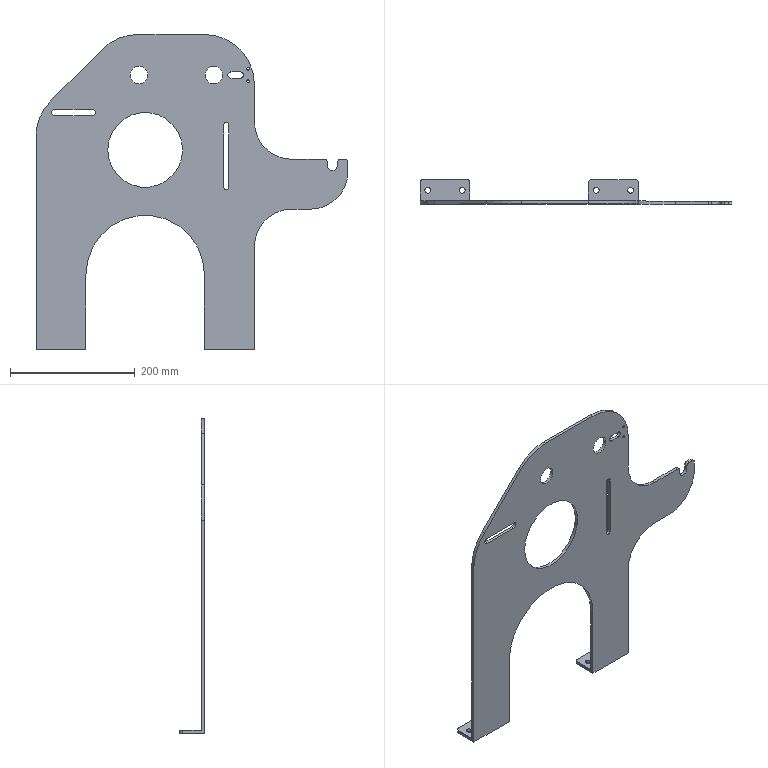Component | SolidWorks | VerticalPlate_Default_ByProcessing-3 | 1 solid | 72 faces | box 500 x 40 x 505 mm | volume 665775 mm3 | cylinder 41 | plane 27 | cone 4 | commonest cylinder face diameters 10 x13 9.225 x8 120 x5 4.2 x4 28 x4 160 x3 8 x2 16 x1
build123d program:
from build123d import *

# Parameters (mm, degrees)
SKETCH1_W                   = 350
SKETCH1_H                   = 500
BOSS_EXTRUDE1_DEPTH         = 2.5
SKETCH2_W                   = 150
SKETCH2_H                   = 80
BOSS_EXTRUDE2_DEPTH         = 5
SKETCH3_W                   = 350
SKETCH3_H                   = 40
BOSS_EXTRUDE3_DEPTH         = 5
CUT_EXTRUDE1_DEPTH          = 415.578
SKETCH6_R                   = 4.09
CUT_EXTRUDE3_DEPTH          = 598.521
SKETCH7_R                   = 60
CUT_EXTRUDE4_DEPTH          = 416.03
CHAMFER1_SIZE               = 130
FILLET2_R                   = 60
FILLET3_R                   = 80
SKETCH8_R                   = 14
CUT_EXTRUDE5_DEPTH          = 415.578
M5_TAPPED_HOLE1_D           = 4.2
M5_TAPPED_HOLE1_CSINK_D     = 5.05
M5_TAPPED_HOLE1_CSINK_ANGLE = 90
FILLET1_R                   = 5
SKETCH11_R                  = 4.613
CUT_EXTRUDE6_DEPTH          = 598.521
FILLET4_R                   = 60


with BuildPart() as part:
    # Sketch1 → Boss-Extrude1 (new, symmetric)
    with BuildSketch(Plane.XY):
        Rectangle(SKETCH1_W, SKETCH1_H)
    extrude(amount=BOSS_EXTRUDE1_DEPTH, both=True)

    # Sketch2 → Boss-Extrude2 (add)
    with BuildSketch(Plane.XY.offset(2.5)):
        with Locations((-250, 10)):
            Rectangle(SKETCH2_W, SKETCH2_H)
    extrude(amount=-BOSS_EXTRUDE2_DEPTH)

    # Sketch3 → Boss-Extrude3 (add)
    with BuildSketch(Plane.XZ.offset(250)):
        with Locations((0, 17.5)):
            Rectangle(SKETCH3_W, SKETCH3_H)
    extrude(amount=BOSS_EXTRUDE3_DEPTH)

    # Sketch4 → Cut-Extrude1 (cut, through all)
    with BuildSketch(Plane.XY.offset(2.5)):
        with BuildLine():
            Line((-292, 60), (-292, 40))
            ThreePointArc((-292, 40), (-300, 32), (-308, 40))
            Line((-308, 40), (-308, 60))
            ThreePointArc((-308, 60), (-300, 68), (-292, 60))
        make_face()
    extrude(amount=-CUT_EXTRUDE1_DEPTH, mode=Mode.SUBTRACT)

    # Sketch6 → Cut-Extrude3 (cut, through all)
    with BuildSketch(Plane(origin=(0, -250, 0), x_dir=(1, 0, 0), z_dir=(0, 1, 0))):
        with Locations(Location((-11.628, -27.97, 0), (0, 0, 270))):
            Circle(SKETCH6_R)
        with Locations(Location((11.628, -27.97, 0), (0, 0, 90))):
            Circle(SKETCH6_R)
    extrude(amount=-CUT_EXTRUDE3_DEPTH, mode=Mode.SUBTRACT)

    # Sketch7 → Cut-Extrude4 (cut, through all)
    with BuildSketch(Plane(origin=(0, 0, -2.5), x_dir=(-1, 0, 0), z_dir=(0, 0, -1))):
        with Locations((0, 65)):
            Circle(SKETCH7_R)
        with BuildLine():
            Line((-95, -255), (95, -255))
            Line((95, -255), (95, -135))
            ThreePointArc((95, -135), (0, -40), (-95, -135))
            Line((-95, -135), (-95, -255))
        make_face()
    extrude(amount=-CUT_EXTRUDE4_DEPTH, mode=Mode.SUBTRACT)

    # Chamfer1
    chamfer1_edges = [part.edges().sort_by_distance(p)[0] for p in [
        (175, 250, 0),
    ]]
    chamfer(chamfer1_edges, length=CHAMFER1_SIZE)

    # Fillet2
    fillet2_edges = [part.edges().sort_by_distance(p)[0] for p in [
        (-175, 50, 0),
    ]]
    fillet(fillet2_edges, radius=FILLET2_R)

    # Fillet3
    fillet3_edges = [part.edges().sort_by_distance(p)[0] for p in [
        (45, 250, 0),
        (175, 120, 0),
        (-175, 250, 0),
    ]]
    fillet(fillet3_edges, radius=FILLET3_R)

    # Sketch8 → Cut-Extrude5 (cut, through all)
    with BuildSketch(Plane.XY.offset(2.5)):
        with Locations((-110, 185)):
            Circle(SKETCH8_R)
        with Locations((10, 185)):
            Circle(SKETCH8_R)
        with BuildLine():
            Line((-152.5, 190), (-137.5, 190))
            ThreePointArc((-137.5, 190), (-132.5, 185), (-137.5, 180))
            Line((-137.5, 180), (-152.5, 180))
            ThreePointArc((-152.5, 180), (-157.5, 185), (-152.5, 190))
        make_face()
        with BuildLine():
            Line((-126, 105), (-126, 5))
            ThreePointArc((-126, 5), (-130, 1), (-134, 5))
            Line((-134, 5), (-134, 105))
            ThreePointArc((-134, 105), (-130, 109), (-126, 105))
        make_face()
        with BuildLine():
            Line((85, 130), (145, 130))
            ThreePointArc((145, 130), (150, 125), (145, 120))
            Line((145, 120), (85, 120))
            ThreePointArc((85, 120), (80, 125), (85, 130))
        make_face()
    extrude(amount=-CUT_EXTRUDE5_DEPTH, mode=Mode.SUBTRACT)

    # M5 Tapped Hole1 (through all)
    with Locations(Plane.XY.offset(2.5)):
        with Locations((-165, 195), (-165, 175)):
            CounterSinkHole(M5_TAPPED_HOLE1_D / 2, M5_TAPPED_HOLE1_CSINK_D / 2, counter_sink_angle=M5_TAPPED_HOLE1_CSINK_ANGLE)

    # Fillet1
    fillet1_edges = [part.edges().sort_by_distance(p)[0] for p in [
        (-325, 50, 0),
        (-175, -252.5, 37.5),
        (175, -252.5, 37.5),
        (-308, 50, 0),
        (-292, 50, 0),
        (95, -252.5, 37.5),
        (-95, -252.5, 37.5),
    ]]
    fillet(fillet1_edges, radius=FILLET1_R)

    # Sketch11 → Cut-Extrude6 (cut, through all)
    with BuildSketch(Plane(origin=(0, -250, 0), x_dir=(1, 0, 0), z_dir=(0, 1, 0))):
        with Locations(Location((-162.627, -20.213, 0), (0, 0, 270))):
            Circle(SKETCH11_R)
        with Locations(Location((-107.373, -20.213, 0), (0, 0, 90))):
            Circle(SKETCH11_R)
        with Locations(Location((107.373, -20.213, 0), (0, 0, 270))):
            Circle(SKETCH11_R)
        with Locations(Location((162.627, -20.213, 0), (0, 0, 90))):
            Circle(SKETCH11_R)
    extrude(amount=-CUT_EXTRUDE6_DEPTH, mode=Mode.SUBTRACT)

    # Fillet4
    fillet4_edges = [part.edges().sort_by_distance(p)[0] for p in [
        (-175, -30, 0),
        (-325, -30, 0),
    ]]
    fillet(fillet4_edges, radius=FILLET4_R)


solid = part.part

# Placed as in the assembly
solid = solid.moved(Location((-145, 142.5, -185), (-90, 0, 180)))